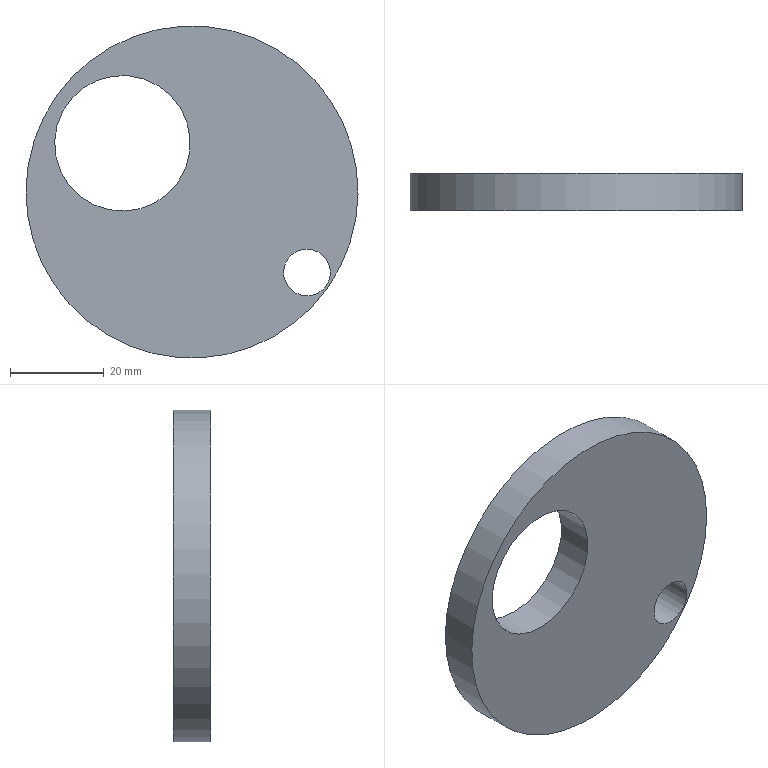Component | NX | ECCENTRIC | 1 solid | 5 faces | box 71 x 8 x 71 mm | volume 25761 mm3 | cylinder 3 | plane 2 | commonest cylinder face diameters 10 x1 71 x1 29 x1
STEP:
#1=CARTESIAN_POINT('',(0.,0.,0.));
#2=DIRECTION('',(0.,0.,1.));
#3=DIRECTION('',(1.,0.,0.));
#4=AXIS2_PLACEMENT_3D('',#1,#2,#3);
#5=CARTESIAN_POINT('',(-122.731,-25.005,87.132));
#6=VERTEX_POINT('',#5);
#7=CARTESIAN_POINT('',(-126.826,-25.005,90.));
#8=DIRECTION('',(0.,-1.,0.));
#9=DIRECTION('',(0.8192,0.,-0.5736));
#10=AXIS2_PLACEMENT_3D('',#7,#8,#9);
#11=CIRCLE('',#10,5.);
#12=CARTESIAN_POINT('',(-126.826,-25.005,90.));
#13=DIRECTION('',(0.,1.,0.));
#14=DIRECTION('',(0.5736,0.,0.8192));
#15=AXIS2_PLACEMENT_3D('',#12,#13,#14);
#16=CYLINDRICAL_SURFACE('',#15,5.);
#17=CARTESIAN_POINT('',(7.854,0.));
#18=DIRECTION('',(-1.,0.));
#19=VECTOR('',#18,1.);
#20=LINE('',#17,#19);
#21=(GEOMETRIC_REPRESENTATION_CONTEXT(2)PARAMETRIC_REPRESENTATION_CONTEXT()REPRESENTATION_CONTEXT('',''));
#22=DEFINITIONAL_REPRESENTATION('',(#20),#21);
#23=PCURVE('',#16,#22);
#24=CARTESIAN_POINT('',(-139.114,-25.005,98.604));
#25=DIRECTION('',(0.,-1.,0.));
#26=DIRECTION('',(-0.5736,0.,-0.8192));
#27=AXIS2_PLACEMENT_3D('',#24,#25,#26);
#28=PLANE('',#27);
#29=CARTESIAN_POINT('',(-0.,15.));
#30=DIRECTION('',(0.,1.));
#31=AXIS2_PLACEMENT_2D('',#29,#30);
#32=CIRCLE('',#31,5.);
#33=(GEOMETRIC_REPRESENTATION_CONTEXT(2)PARAMETRIC_REPRESENTATION_CONTEXT()REPRESENTATION_CONTEXT('',''));
#34=DEFINITIONAL_REPRESENTATION('',(#32),#33);
#35=PCURVE('',#28,#34);
#36=SURFACE_CURVE('',#11,(#23,#35),.PCURVE_S1.);
#37=EDGE_CURVE('',#6,#6,#36,.T.);
#38=ORIENTED_EDGE('',*,*,#37,.F.);
#39=CARTESIAN_POINT('',(-122.731,-17.005,87.132));
#40=VERTEX_POINT('',#39);
#41=CARTESIAN_POINT('',(-122.731,-25.005,87.132));
#42=CARTESIAN_POINT('',(-122.731,-17.005,87.132));
#43=B_SPLINE_CURVE_WITH_KNOTS('',1,(#41,#42),.UNSPECIFIED.,.F.,.F.,(2,2),(0.,8.),.PIECEWISE_BEZIER_KNOTS.);
#44=CARTESIAN_POINT('',(7.854,0.));
#45=DIRECTION('',(0.,1.));
#46=VECTOR('',#45,1.);
#47=LINE('',#44,#46);
#48=(GEOMETRIC_REPRESENTATION_CONTEXT(2)PARAMETRIC_REPRESENTATION_CONTEXT()REPRESENTATION_CONTEXT('',''));
#49=DEFINITIONAL_REPRESENTATION('',(#47),#48);
#50=PCURVE('',#16,#49);
#51=CARTESIAN_POINT('',(1.571,0.));
#52=DIRECTION('',(0.,1.));
#53=VECTOR('',#52,1.);
#54=LINE('',#51,#53);
#55=(GEOMETRIC_REPRESENTATION_CONTEXT(2)PARAMETRIC_REPRESENTATION_CONTEXT()REPRESENTATION_CONTEXT('',''));
#56=DEFINITIONAL_REPRESENTATION('',(#54),#55);
#57=PCURVE('',#16,#56);
#58=SEAM_CURVE('',#43,(#50,#57),.PCURVE_S1.);
#59=EDGE_CURVE('',#6,#40,#58,.T.);
#60=ORIENTED_EDGE('',*,*,#59,.T.);
#61=CARTESIAN_POINT('',(-126.826,-17.005,90.));
#62=DIRECTION('',(0.,-1.,0.));
#63=DIRECTION('',(0.8192,0.,-0.5736));
#64=AXIS2_PLACEMENT_3D('',#61,#62,#63);
#65=CIRCLE('',#64,5.);
#66=CARTESIAN_POINT('',(7.854,8.));
#67=DIRECTION('',(-1.,0.));
#68=VECTOR('',#67,1.);
#69=LINE('',#66,#68);
#70=(GEOMETRIC_REPRESENTATION_CONTEXT(2)PARAMETRIC_REPRESENTATION_CONTEXT()REPRESENTATION_CONTEXT('',''));
#71=DEFINITIONAL_REPRESENTATION('',(#69),#70);
#72=PCURVE('',#16,#71);
#73=CARTESIAN_POINT('',(-139.114,-17.005,98.604));
#74=DIRECTION('',(0.,-1.,0.));
#75=DIRECTION('',(-0.5736,0.,-0.8192));
#76=AXIS2_PLACEMENT_3D('',#73,#74,#75);
#77=PLANE('',#76);
#78=CARTESIAN_POINT('',(-0.,15.));
#79=DIRECTION('',(0.,1.));
#80=AXIS2_PLACEMENT_2D('',#78,#79);
#81=CIRCLE('',#80,5.);
#82=(GEOMETRIC_REPRESENTATION_CONTEXT(2)PARAMETRIC_REPRESENTATION_CONTEXT()REPRESENTATION_CONTEXT('',''));
#83=DEFINITIONAL_REPRESENTATION('',(#81),#82);
#84=PCURVE('',#77,#83);
#85=SURFACE_CURVE('',#65,(#72,#84),.PCURVE_S1.);
#86=EDGE_CURVE('',#40,#40,#85,.T.);
#87=ORIENTED_EDGE('',*,*,#86,.T.);
#88=ORIENTED_EDGE('',*,*,#59,.F.);
#89=EDGE_LOOP('',(#38,#60,#87,#88));
#90=FACE_BOUND('',#89,.F.);
#91=ADVANCED_FACE('',(#90),#16,.F.);
#92=CARTESIAN_POINT('',(-122.321,-25.005,86.845));
#93=VERTEX_POINT('',#92);
#94=CARTESIAN_POINT('',(-151.401,-25.005,107.207));
#95=DIRECTION('',(0.,-1.,0.));
#96=DIRECTION('',(0.8192,0.,-0.5736));
#97=AXIS2_PLACEMENT_3D('',#94,#95,#96);
#98=CIRCLE('',#97,35.5);
#99=CARTESIAN_POINT('',(-151.401,-25.005,107.207));
#100=DIRECTION('',(0.,1.,0.));
#101=DIRECTION('',(0.5736,0.,0.8192));
#102=AXIS2_PLACEMENT_3D('',#99,#100,#101);
#103=CYLINDRICAL_SURFACE('',#102,35.5);
#104=CARTESIAN_POINT('',(7.854,0.));
#105=DIRECTION('',(-1.,0.));
#106=VECTOR('',#105,1.);
#107=LINE('',#104,#106);
#108=(GEOMETRIC_REPRESENTATION_CONTEXT(2)PARAMETRIC_REPRESENTATION_CONTEXT()REPRESENTATION_CONTEXT('',''));
#109=DEFINITIONAL_REPRESENTATION('',(#107),#108);
#110=PCURVE('',#103,#109);
#111=CARTESIAN_POINT('',(0.,-15.));
#112=DIRECTION('',(0.,1.));
#113=AXIS2_PLACEMENT_2D('',#111,#112);
#114=CIRCLE('',#113,35.5);
#115=(GEOMETRIC_REPRESENTATION_CONTEXT(2)PARAMETRIC_REPRESENTATION_CONTEXT()REPRESENTATION_CONTEXT('',''));
#116=DEFINITIONAL_REPRESENTATION('',(#114),#115);
#117=PCURVE('',#28,#116);
#118=SURFACE_CURVE('',#98,(#110,#117),.PCURVE_S1.);
#119=EDGE_CURVE('',#93,#93,#118,.T.);
#120=ORIENTED_EDGE('',*,*,#119,.F.);
#121=CARTESIAN_POINT('',(-122.321,-17.005,86.845));
#122=VERTEX_POINT('',#121);
#123=CARTESIAN_POINT('',(-122.321,-25.005,86.845));
#124=CARTESIAN_POINT('',(-122.321,-17.005,86.845));
#125=B_SPLINE_CURVE_WITH_KNOTS('',1,(#123,#124),.UNSPECIFIED.,.F.,.F.,(2,2),(0.,8.),.PIECEWISE_BEZIER_KNOTS.);
#126=CARTESIAN_POINT('',(7.854,0.));
#127=DIRECTION('',(0.,1.));
#128=VECTOR('',#127,1.);
#129=LINE('',#126,#128);
#130=(GEOMETRIC_REPRESENTATION_CONTEXT(2)PARAMETRIC_REPRESENTATION_CONTEXT()REPRESENTATION_CONTEXT('',''));
#131=DEFINITIONAL_REPRESENTATION('',(#129),#130);
#132=PCURVE('',#103,#131);
#133=CARTESIAN_POINT('',(1.571,0.));
#134=DIRECTION('',(0.,1.));
#135=VECTOR('',#134,1.);
#136=LINE('',#133,#135);
#137=(GEOMETRIC_REPRESENTATION_CONTEXT(2)PARAMETRIC_REPRESENTATION_CONTEXT()REPRESENTATION_CONTEXT('',''));
#138=DEFINITIONAL_REPRESENTATION('',(#136),#137);
#139=PCURVE('',#103,#138);
#140=SEAM_CURVE('',#125,(#132,#139),.PCURVE_S1.);
#141=EDGE_CURVE('',#93,#122,#140,.T.);
#142=ORIENTED_EDGE('',*,*,#141,.T.);
#143=CARTESIAN_POINT('',(-151.401,-17.005,107.207));
#144=DIRECTION('',(0.,-1.,0.));
#145=DIRECTION('',(0.8192,0.,-0.5736));
#146=AXIS2_PLACEMENT_3D('',#143,#144,#145);
#147=CIRCLE('',#146,35.5);
#148=CARTESIAN_POINT('',(7.854,8.));
#149=DIRECTION('',(-1.,0.));
#150=VECTOR('',#149,1.);
#151=LINE('',#148,#150);
#152=(GEOMETRIC_REPRESENTATION_CONTEXT(2)PARAMETRIC_REPRESENTATION_CONTEXT()REPRESENTATION_CONTEXT('',''));
#153=DEFINITIONAL_REPRESENTATION('',(#151),#152);
#154=PCURVE('',#103,#153);
#155=CARTESIAN_POINT('',(0.,-15.));
#156=DIRECTION('',(0.,1.));
#157=AXIS2_PLACEMENT_2D('',#155,#156);
#158=CIRCLE('',#157,35.5);
#159=(GEOMETRIC_REPRESENTATION_CONTEXT(2)PARAMETRIC_REPRESENTATION_CONTEXT()REPRESENTATION_CONTEXT('',''));
#160=DEFINITIONAL_REPRESENTATION('',(#158),#159);
#161=PCURVE('',#77,#160);
#162=SURFACE_CURVE('',#147,(#154,#161),.PCURVE_S1.);
#163=EDGE_CURVE('',#122,#122,#162,.T.);
#164=ORIENTED_EDGE('',*,*,#163,.T.);
#165=ORIENTED_EDGE('',*,*,#141,.F.);
#166=EDGE_LOOP('',(#120,#142,#164,#165));
#167=FACE_BOUND('',#166,.T.);
#168=ADVANCED_FACE('',(#167),#103,.T.);
#169=CARTESIAN_POINT('',(-154.396,-25.005,109.305));
#170=VERTEX_POINT('',#169);
#171=CARTESIAN_POINT('',(-166.274,-25.005,117.621));
#172=DIRECTION('',(0.,-1.,0.));
#173=DIRECTION('',(0.8192,0.,-0.5736));
#174=AXIS2_PLACEMENT_3D('',#171,#172,#173);
#175=CIRCLE('',#174,14.5);
#176=CARTESIAN_POINT('',(-166.274,-25.005,117.621));
#177=DIRECTION('',(0.,1.,0.));
#178=DIRECTION('',(0.5736,0.,0.8192));
#179=AXIS2_PLACEMENT_3D('',#176,#177,#178);
#180=CYLINDRICAL_SURFACE('',#179,14.5);
#181=CARTESIAN_POINT('',(7.854,0.));
#182=DIRECTION('',(-1.,0.));
#183=VECTOR('',#182,1.);
#184=LINE('',#181,#183);
#185=(GEOMETRIC_REPRESENTATION_CONTEXT(2)PARAMETRIC_REPRESENTATION_CONTEXT()REPRESENTATION_CONTEXT('',''));
#186=DEFINITIONAL_REPRESENTATION('',(#184),#185);
#187=PCURVE('',#180,#186);
#188=CARTESIAN_POINT('',(0.,-33.156));
#189=DIRECTION('',(0.,1.));
#190=AXIS2_PLACEMENT_2D('',#188,#189);
#191=CIRCLE('',#190,14.5);
#192=(GEOMETRIC_REPRESENTATION_CONTEXT(2)PARAMETRIC_REPRESENTATION_CONTEXT()REPRESENTATION_CONTEXT('',''));
#193=DEFINITIONAL_REPRESENTATION('',(#191),#192);
#194=PCURVE('',#28,#193);
#195=SURFACE_CURVE('',#175,(#187,#194),.PCURVE_S1.);
#196=EDGE_CURVE('',#170,#170,#195,.T.);
#197=ORIENTED_EDGE('',*,*,#196,.F.);
#198=CARTESIAN_POINT('',(-154.396,-17.005,109.305));
#199=VERTEX_POINT('',#198);
#200=CARTESIAN_POINT('',(-154.396,-25.005,109.305));
#201=CARTESIAN_POINT('',(-154.396,-17.005,109.305));
#202=B_SPLINE_CURVE_WITH_KNOTS('',1,(#200,#201),.UNSPECIFIED.,.F.,.F.,(2,2),(0.,8.),.PIECEWISE_BEZIER_KNOTS.);
#203=CARTESIAN_POINT('',(7.854,0.));
#204=DIRECTION('',(0.,1.));
#205=VECTOR('',#204,1.);
#206=LINE('',#203,#205);
#207=(GEOMETRIC_REPRESENTATION_CONTEXT(2)PARAMETRIC_REPRESENTATION_CONTEXT()REPRESENTATION_CONTEXT('',''));
#208=DEFINITIONAL_REPRESENTATION('',(#206),#207);
#209=PCURVE('',#180,#208);
#210=CARTESIAN_POINT('',(1.571,0.));
#211=DIRECTION('',(0.,1.));
#212=VECTOR('',#211,1.);
#213=LINE('',#210,#212);
#214=(GEOMETRIC_REPRESENTATION_CONTEXT(2)PARAMETRIC_REPRESENTATION_CONTEXT()REPRESENTATION_CONTEXT('',''));
#215=DEFINITIONAL_REPRESENTATION('',(#213),#214);
#216=PCURVE('',#180,#215);
#217=SEAM_CURVE('',#202,(#209,#216),.PCURVE_S1.);
#218=EDGE_CURVE('',#170,#199,#217,.T.);
#219=ORIENTED_EDGE('',*,*,#218,.T.);
#220=CARTESIAN_POINT('',(-166.274,-17.005,117.621));
#221=DIRECTION('',(0.,-1.,0.));
#222=DIRECTION('',(0.8192,0.,-0.5736));
#223=AXIS2_PLACEMENT_3D('',#220,#221,#222);
#224=CIRCLE('',#223,14.5);
#225=CARTESIAN_POINT('',(7.854,8.));
#226=DIRECTION('',(-1.,0.));
#227=VECTOR('',#226,1.);
#228=LINE('',#225,#227);
#229=(GEOMETRIC_REPRESENTATION_CONTEXT(2)PARAMETRIC_REPRESENTATION_CONTEXT()REPRESENTATION_CONTEXT('',''));
#230=DEFINITIONAL_REPRESENTATION('',(#228),#229);
#231=PCURVE('',#180,#230);
#232=CARTESIAN_POINT('',(0.,-33.156));
#233=DIRECTION('',(0.,1.));
#234=AXIS2_PLACEMENT_2D('',#232,#233);
#235=CIRCLE('',#234,14.5);
#236=(GEOMETRIC_REPRESENTATION_CONTEXT(2)PARAMETRIC_REPRESENTATION_CONTEXT()REPRESENTATION_CONTEXT('',''));
#237=DEFINITIONAL_REPRESENTATION('',(#235),#236);
#238=PCURVE('',#77,#237);
#239=SURFACE_CURVE('',#224,(#231,#238),.PCURVE_S1.);
#240=EDGE_CURVE('',#199,#199,#239,.T.);
#241=ORIENTED_EDGE('',*,*,#240,.T.);
#242=ORIENTED_EDGE('',*,*,#218,.F.);
#243=EDGE_LOOP('',(#197,#219,#241,#242));
#244=FACE_BOUND('',#243,.F.);
#245=ADVANCED_FACE('',(#244),#180,.F.);
#246=ORIENTED_EDGE('',*,*,#119,.T.);
#247=EDGE_LOOP('',(#246));
#248=FACE_BOUND('',#247,.T.);
#249=ORIENTED_EDGE('',*,*,#37,.F.);
#250=EDGE_LOOP('',(#249));
#251=FACE_BOUND('',#250,.T.);
#252=ORIENTED_EDGE('',*,*,#196,.F.);
#253=EDGE_LOOP('',(#252));
#254=FACE_BOUND('',#253,.T.);
#255=ADVANCED_FACE('',(#248,#251,#254),#28,.T.);
#256=ORIENTED_EDGE('',*,*,#163,.F.);
#257=EDGE_LOOP('',(#256));
#258=FACE_BOUND('',#257,.T.);
#259=ORIENTED_EDGE('',*,*,#86,.T.);
#260=EDGE_LOOP('',(#259));
#261=FACE_BOUND('',#260,.T.);
#262=ORIENTED_EDGE('',*,*,#240,.T.);
#263=EDGE_LOOP('',(#262));
#264=FACE_BOUND('',#263,.T.);
#265=ADVANCED_FACE('',(#258,#261,#264),#77,.F.);
#266=CLOSED_SHELL('',(#91,#168,#245,#255,#265));
#267=MANIFOLD_SOLID_BREP('',#266);
#268=(LENGTH_UNIT()NAMED_UNIT(*)SI_UNIT(.MILLI.,.METRE.));
#269=UNCERTAINTY_MEASURE_WITH_UNIT(LENGTH_MEASURE(0.00001),#268,'','');
#270=(NAMED_UNIT(*)PLANE_ANGLE_UNIT()SI_UNIT($,.RADIAN.));
#271=(NAMED_UNIT(*)SI_UNIT($,.STERADIAN.)SOLID_ANGLE_UNIT());
#272=(GEOMETRIC_REPRESENTATION_CONTEXT(3)GLOBAL_UNCERTAINTY_ASSIGNED_CONTEXT((#269))GLOBAL_UNIT_ASSIGNED_CONTEXT((#268,#270,#271))REPRESENTATION_CONTEXT('',''));
#273=ADVANCED_BREP_SHAPE_REPRESENTATION('',(#4,#267),#272);